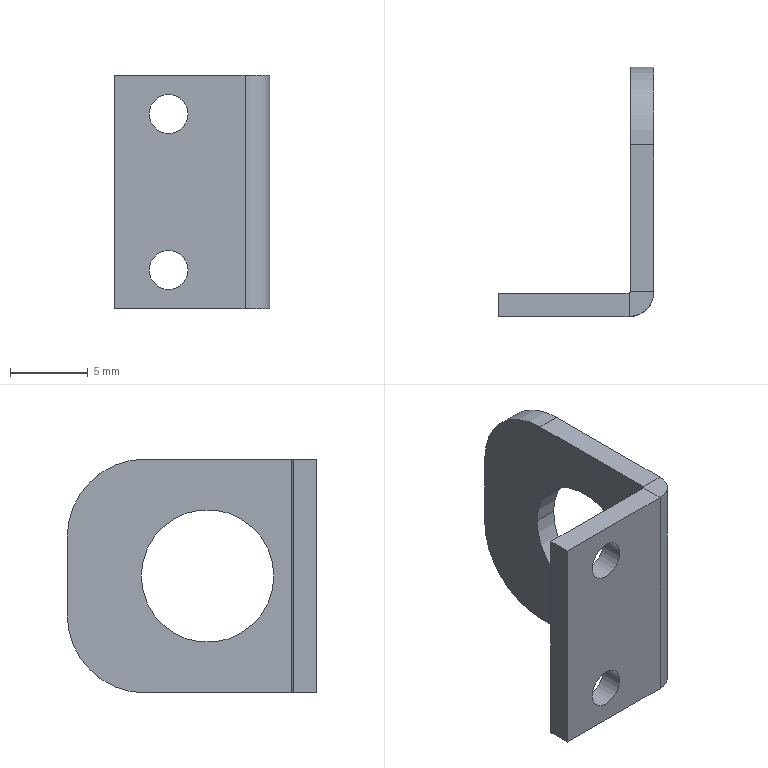Component | SolidWorks | FrontDoorAssembly-1_FrontDoorWelding-1_CustomLockBarGuidePlate-1 | 1 solid | 22 faces | box 10 x 16 x 15 mm | volume 427 mm3 | plane 12 | cylinder 10 | commonest cylinder face diameters 2.5 x4 8.5 x2 10 x2 3.2 x1 0.2 x1
STEP:
#1=CARTESIAN_POINT('',(-37.852,-11.035,14.951));
#2=VERTEX_POINT('',#1);
#3=CARTESIAN_POINT('',(-37.753,-11.035,14.951));
#4=VERTEX_POINT('',#3);
#5=CARTESIAN_POINT('',(-37.803,-11.035,14.951));
#6=DIRECTION('',(-0.,1.,-0.));
#7=DIRECTION('',(1.,0.,0.));
#8=AXIS2_PLACEMENT_3D('',#5,#6,#7);
#9=CIRCLE('',#8,0.04921);
#10=EDGE_CURVE('',#2,#4,#9,.T.);
#11=ORIENTED_EDGE('',*,*,#10,.F.);
#12=CARTESIAN_POINT('',(-37.852,-10.976,14.951));
#13=VERTEX_POINT('',#12);
#14=CARTESIAN_POINT('',(-37.852,-11.37,14.951));
#15=DIRECTION('',(-0.,1.,-0.));
#16=VECTOR('',#15,39.37);
#17=LINE('',#14,#16);
#18=EDGE_CURVE('',#2,#13,#17,.T.);
#19=ORIENTED_EDGE('',*,*,#18,.T.);
#20=CARTESIAN_POINT('',(-37.753,-10.976,14.951));
#21=VERTEX_POINT('',#20);
#22=CARTESIAN_POINT('',(-37.803,-10.976,14.951));
#23=DIRECTION('',(-0.,1.,-0.));
#24=DIRECTION('',(-1.,0.,0.));
#25=AXIS2_PLACEMENT_3D('',#22,#23,#24);
#26=CIRCLE('',#25,0.04921);
#27=EDGE_CURVE('',#13,#21,#26,.T.);
#28=ORIENTED_EDGE('',*,*,#27,.T.);
#29=CARTESIAN_POINT('',(-37.753,-11.37,14.951));
#30=DIRECTION('',(-0.,1.,-0.));
#31=VECTOR('',#30,39.37);
#32=LINE('',#29,#31);
#33=EDGE_CURVE('',#4,#21,#32,.T.);
#34=ORIENTED_EDGE('',*,*,#33,.F.);
#35=EDGE_LOOP('',(#11,#19,#28,#34));
#36=FACE_OUTER_BOUND('',#35,.T.);
#37=CARTESIAN_POINT('',(-37.803,-11.37,14.951));
#38=DIRECTION('',(-0.,1.,-0.));
#39=DIRECTION('',(1.,0.,0.));
#40=AXIS2_PLACEMENT_3D('',#37,#38,#39);
#41=CYLINDRICAL_SURFACE('',#40,0.04921);
#42=ADVANCED_FACE('',(#36),#41,.F.);
#43=CARTESIAN_POINT('',(-37.852,-11.035,14.557));
#44=VERTEX_POINT('',#43);
#45=CARTESIAN_POINT('',(-37.753,-11.035,14.557));
#46=VERTEX_POINT('',#45);
#47=CARTESIAN_POINT('',(-37.803,-11.035,14.557));
#48=DIRECTION('',(-0.,1.,-0.));
#49=DIRECTION('',(1.,0.,0.));
#50=AXIS2_PLACEMENT_3D('',#47,#48,#49);
#51=CIRCLE('',#50,0.04921);
#52=EDGE_CURVE('',#44,#46,#51,.T.);
#53=ORIENTED_EDGE('',*,*,#52,.F.);
#54=CARTESIAN_POINT('',(-37.852,-10.976,14.557));
#55=VERTEX_POINT('',#54);
#56=CARTESIAN_POINT('',(-37.852,-11.37,14.557));
#57=DIRECTION('',(-0.,1.,-0.));
#58=VECTOR('',#57,39.37);
#59=LINE('',#56,#58);
#60=EDGE_CURVE('',#44,#55,#59,.T.);
#61=ORIENTED_EDGE('',*,*,#60,.T.);
#62=CARTESIAN_POINT('',(-37.753,-10.976,14.557));
#63=VERTEX_POINT('',#62);
#64=CARTESIAN_POINT('',(-37.803,-10.976,14.557));
#65=DIRECTION('',(-0.,1.,-0.));
#66=DIRECTION('',(1.,0.,0.));
#67=AXIS2_PLACEMENT_3D('',#64,#65,#66);
#68=CIRCLE('',#67,0.04921);
#69=EDGE_CURVE('',#55,#63,#68,.T.);
#70=ORIENTED_EDGE('',*,*,#69,.T.);
#71=CARTESIAN_POINT('',(-37.753,-11.37,14.557));
#72=DIRECTION('',(-0.,1.,-0.));
#73=VECTOR('',#72,39.37);
#74=LINE('',#71,#73);
#75=EDGE_CURVE('',#46,#63,#74,.T.);
#76=ORIENTED_EDGE('',*,*,#75,.F.);
#77=EDGE_LOOP('',(#53,#61,#70,#76));
#78=FACE_OUTER_BOUND('',#77,.T.);
#79=CARTESIAN_POINT('',(-37.803,-11.37,14.557));
#80=DIRECTION('',(-0.,1.,-0.));
#81=DIRECTION('',(1.,0.,0.));
#82=AXIS2_PLACEMENT_3D('',#79,#80,#81);
#83=CYLINDRICAL_SURFACE('',#82,0.04921);
#84=ADVANCED_FACE('',(#78),#83,.F.);
#85=CARTESIAN_POINT('',(-37.547,-10.927,14.754));
#86=VERTEX_POINT('',#85);
#87=CARTESIAN_POINT('',(-37.547,-10.592,14.754));
#88=VERTEX_POINT('',#87);
#89=CARTESIAN_POINT('',(-37.547,-10.76,14.754));
#90=DIRECTION('',(-1.,0.,0.));
#91=DIRECTION('',(0.,1.,0.));
#92=AXIS2_PLACEMENT_3D('',#89,#90,#91);
#93=CIRCLE('',#92,0.1673);
#94=EDGE_CURVE('',#86,#88,#93,.T.);
#95=ORIENTED_EDGE('',*,*,#94,.F.);
#96=CARTESIAN_POINT('',(-37.606,-10.927,14.754));
#97=VERTEX_POINT('',#96);
#98=CARTESIAN_POINT('',(-37.212,-10.927,14.754));
#99=DIRECTION('',(-1.,0.,0.));
#100=VECTOR('',#99,39.37);
#101=LINE('',#98,#100);
#102=EDGE_CURVE('',#86,#97,#101,.T.);
#103=ORIENTED_EDGE('',*,*,#102,.T.);
#104=CARTESIAN_POINT('',(-37.606,-10.592,14.754));
#105=VERTEX_POINT('',#104);
#106=CARTESIAN_POINT('',(-37.606,-10.76,14.754));
#107=DIRECTION('',(-1.,0.,0.));
#108=DIRECTION('',(0.,1.,0.));
#109=AXIS2_PLACEMENT_3D('',#106,#107,#108);
#110=CIRCLE('',#109,0.1673);
#111=EDGE_CURVE('',#97,#105,#110,.T.);
#112=ORIENTED_EDGE('',*,*,#111,.T.);
#113=CARTESIAN_POINT('',(-37.212,-10.592,14.754));
#114=DIRECTION('',(-1.,0.,0.));
#115=VECTOR('',#114,39.37);
#116=LINE('',#113,#115);
#117=EDGE_CURVE('',#88,#105,#116,.T.);
#118=ORIENTED_EDGE('',*,*,#117,.F.);
#119=EDGE_LOOP('',(#95,#103,#112,#118));
#120=FACE_OUTER_BOUND('',#119,.T.);
#121=CARTESIAN_POINT('',(-37.212,-10.76,14.754));
#122=DIRECTION('',(-1.,0.,0.));
#123=DIRECTION('',(0.,1.,0.));
#124=AXIS2_PLACEMENT_3D('',#121,#122,#123);
#125=CYLINDRICAL_SURFACE('',#124,0.1673);
#126=ADVANCED_FACE('',(#120),#125,.F.);
#127=CARTESIAN_POINT('',(-37.547,-10.972,15.049));
#128=VERTEX_POINT('',#127);
#129=CARTESIAN_POINT('',(-37.547,-10.602,15.049));
#130=VERTEX_POINT('',#129);
#131=CARTESIAN_POINT('',(-37.547,-10.405,15.049));
#132=DIRECTION('',(0.,1.,-0.));
#133=VECTOR('',#132,39.37);
#134=LINE('',#131,#133);
#135=EDGE_CURVE('',#128,#130,#134,.T.);
#136=ORIENTED_EDGE('',*,*,#135,.T.);
#137=CARTESIAN_POINT('',(-37.606,-10.602,15.049));
#138=VERTEX_POINT('',#137);
#139=CARTESIAN_POINT('',(-37.547,-10.602,15.049));
#140=DIRECTION('',(-1.,0.,0.));
#141=VECTOR('',#140,39.37);
#142=LINE('',#139,#141);
#143=EDGE_CURVE('',#130,#138,#142,.T.);
#144=ORIENTED_EDGE('',*,*,#143,.T.);
#145=CARTESIAN_POINT('',(-37.606,-10.972,15.049));
#146=VERTEX_POINT('',#145);
#147=CARTESIAN_POINT('',(-37.606,-10.405,15.049));
#148=DIRECTION('',(0.,1.,-0.));
#149=VECTOR('',#148,39.37);
#150=LINE('',#147,#149);
#151=EDGE_CURVE('',#146,#138,#150,.T.);
#152=ORIENTED_EDGE('',*,*,#151,.F.);
#153=CARTESIAN_POINT('',(-37.606,-10.972,15.049));
#154=DIRECTION('',(1.,-0.,-0.));
#155=VECTOR('',#154,39.37);
#156=LINE('',#153,#155);
#157=EDGE_CURVE('',#146,#128,#156,.T.);
#158=ORIENTED_EDGE('',*,*,#157,.T.);
#159=EDGE_LOOP('',(#136,#144,#152,#158));
#160=FACE_OUTER_BOUND('',#159,.T.);
#161=CARTESIAN_POINT('',(-37.547,-10.405,15.049));
#162=DIRECTION('',(0.,0.,1.));
#163=DIRECTION('',(0.,1.,-0.));
#164=AXIS2_PLACEMENT_3D('',#161,#162,#163);
#165=PLANE('',#164);
#166=ADVANCED_FACE('',(#160),#165,.T.);
#167=CARTESIAN_POINT('',(-37.547,-10.76,14.754));
#168=DIRECTION('',(-1.,0.,0.));
#169=DIRECTION('',(0.,1.,0.));
#170=AXIS2_PLACEMENT_3D('',#167,#168,#169);
#171=CIRCLE('',#170,0.1673);
#172=EDGE_CURVE('',#88,#86,#171,.T.);
#173=ORIENTED_EDGE('',*,*,#172,.T.);
#174=ORIENTED_EDGE('',*,*,#94,.T.);
#175=EDGE_LOOP('',(#173,#174));
#176=FACE_BOUND('',#175,.T.);
#177=CARTESIAN_POINT('',(-37.547,-10.405,14.853));
#178=VERTEX_POINT('',#177);
#179=CARTESIAN_POINT('',(-37.547,-10.405,14.656));
#180=VERTEX_POINT('',#179);
#181=CARTESIAN_POINT('',(-37.547,-10.405,15.049));
#182=DIRECTION('',(-0.,-0.,-1.));
#183=VECTOR('',#182,39.37);
#184=LINE('',#181,#183);
#185=EDGE_CURVE('',#178,#180,#184,.T.);
#186=ORIENTED_EDGE('',*,*,#185,.F.);
#187=CARTESIAN_POINT('',(-37.547,-10.602,14.853));
#188=DIRECTION('',(1.,-0.,-0.));
#189=DIRECTION('',(0.,1.,0.));
#190=AXIS2_PLACEMENT_3D('',#187,#188,#189);
#191=CIRCLE('',#190,0.1969);
#192=EDGE_CURVE('',#178,#130,#191,.T.);
#193=ORIENTED_EDGE('',*,*,#192,.T.);
#194=ORIENTED_EDGE('',*,*,#135,.F.);
#195=CARTESIAN_POINT('',(-37.547,-10.972,14.459));
#196=VERTEX_POINT('',#195);
#197=CARTESIAN_POINT('',(-37.547,-10.972,15.049));
#198=DIRECTION('',(-0.,-0.,-1.));
#199=VECTOR('',#198,39.37);
#200=LINE('',#197,#199);
#201=EDGE_CURVE('',#128,#196,#200,.T.);
#202=ORIENTED_EDGE('',*,*,#201,.T.);
#203=CARTESIAN_POINT('',(-37.547,-10.602,14.459));
#204=VERTEX_POINT('',#203);
#205=CARTESIAN_POINT('',(-37.547,-10.405,14.459));
#206=DIRECTION('',(-0.,-1.,0.));
#207=VECTOR('',#206,39.37);
#208=LINE('',#205,#207);
#209=EDGE_CURVE('',#204,#196,#208,.T.);
#210=ORIENTED_EDGE('',*,*,#209,.F.);
#211=CARTESIAN_POINT('',(-37.547,-10.602,14.656));
#212=DIRECTION('',(1.,-0.,-0.));
#213=DIRECTION('',(0.,1.,0.));
#214=AXIS2_PLACEMENT_3D('',#211,#212,#213);
#215=CIRCLE('',#214,0.1969);
#216=EDGE_CURVE('',#204,#180,#215,.T.);
#217=ORIENTED_EDGE('',*,*,#216,.T.);
#218=EDGE_LOOP('',(#186,#193,#194,#202,#210,#217));
#219=FACE_OUTER_BOUND('',#218,.T.);
#220=CARTESIAN_POINT('',(-37.547,-10.72,14.754));
#221=DIRECTION('',(-1.,0.,0.));
#222=DIRECTION('',(0.,1.,-0.));
#223=AXIS2_PLACEMENT_3D('',#220,#221,#222);
#224=PLANE('',#223);
#225=ADVANCED_FACE('',(#176,#219),#224,.F.);
#226=CARTESIAN_POINT('',(-37.606,-10.76,14.754));
#227=DIRECTION('',(-1.,0.,0.));
#228=DIRECTION('',(0.,1.,0.));
#229=AXIS2_PLACEMENT_3D('',#226,#227,#228);
#230=CIRCLE('',#229,0.1673);
#231=EDGE_CURVE('',#105,#97,#230,.T.);
#232=ORIENTED_EDGE('',*,*,#231,.F.);
#233=ORIENTED_EDGE('',*,*,#111,.F.);
#234=EDGE_LOOP('',(#232,#233));
#235=FACE_BOUND('',#234,.T.);
#236=ORIENTED_EDGE('',*,*,#151,.T.);
#237=CARTESIAN_POINT('',(-37.606,-10.405,14.853));
#238=VERTEX_POINT('',#237);
#239=CARTESIAN_POINT('',(-37.606,-10.602,14.853));
#240=DIRECTION('',(-1.,0.,0.));
#241=DIRECTION('',(0.,1.,0.));
#242=AXIS2_PLACEMENT_3D('',#239,#240,#241);
#243=CIRCLE('',#242,0.1969);
#244=EDGE_CURVE('',#138,#238,#243,.T.);
#245=ORIENTED_EDGE('',*,*,#244,.T.);
#246=CARTESIAN_POINT('',(-37.606,-10.405,14.656));
#247=VERTEX_POINT('',#246);
#248=CARTESIAN_POINT('',(-37.606,-10.405,15.049));
#249=DIRECTION('',(-0.,-0.,-1.));
#250=VECTOR('',#249,39.37);
#251=LINE('',#248,#250);
#252=EDGE_CURVE('',#238,#247,#251,.T.);
#253=ORIENTED_EDGE('',*,*,#252,.T.);
#254=CARTESIAN_POINT('',(-37.606,-10.602,14.459));
#255=VERTEX_POINT('',#254);
#256=CARTESIAN_POINT('',(-37.606,-10.602,14.656));
#257=DIRECTION('',(-1.,0.,0.));
#258=DIRECTION('',(0.,1.,0.));
#259=AXIS2_PLACEMENT_3D('',#256,#257,#258);
#260=CIRCLE('',#259,0.1969);
#261=EDGE_CURVE('',#247,#255,#260,.T.);
#262=ORIENTED_EDGE('',*,*,#261,.T.);
#263=CARTESIAN_POINT('',(-37.606,-10.972,14.459));
#264=VERTEX_POINT('',#263);
#265=CARTESIAN_POINT('',(-37.606,-10.405,14.459));
#266=DIRECTION('',(-0.,-1.,0.));
#267=VECTOR('',#266,39.37);
#268=LINE('',#265,#267);
#269=EDGE_CURVE('',#255,#264,#268,.T.);
#270=ORIENTED_EDGE('',*,*,#269,.T.);
#271=CARTESIAN_POINT('',(-37.606,-10.972,15.049));
#272=DIRECTION('',(-0.,-0.,-1.));
#273=VECTOR('',#272,39.37);
#274=LINE('',#271,#273);
#275=EDGE_CURVE('',#146,#264,#274,.T.);
#276=ORIENTED_EDGE('',*,*,#275,.F.);
#277=EDGE_LOOP('',(#236,#245,#253,#262,#270,#276));
#278=FACE_OUTER_BOUND('',#277,.T.);
#279=CARTESIAN_POINT('',(-37.606,-10.72,14.754));
#280=DIRECTION('',(-1.,0.,0.));
#281=DIRECTION('',(0.,1.,-0.));
#282=AXIS2_PLACEMENT_3D('',#279,#280,#281);
#283=PLANE('',#282);
#284=ADVANCED_FACE('',(#235,#278),#283,.T.);
#285=ORIENTED_EDGE('',*,*,#269,.F.);
#286=CARTESIAN_POINT('',(-37.547,-10.602,14.459));
#287=DIRECTION('',(1.,-0.,-0.));
#288=VECTOR('',#287,39.37);
#289=LINE('',#286,#288);
#290=EDGE_CURVE('',#255,#204,#289,.T.);
#291=ORIENTED_EDGE('',*,*,#290,.T.);
#292=ORIENTED_EDGE('',*,*,#209,.T.);
#293=CARTESIAN_POINT('',(-37.606,-10.972,14.459));
#294=DIRECTION('',(1.,-0.,-0.));
#295=VECTOR('',#294,39.37);
#296=LINE('',#293,#295);
#297=EDGE_CURVE('',#264,#196,#296,.T.);
#298=ORIENTED_EDGE('',*,*,#297,.F.);
#299=EDGE_LOOP('',(#285,#291,#292,#298));
#300=FACE_OUTER_BOUND('',#299,.T.);
#301=CARTESIAN_POINT('',(-37.547,-10.405,14.459));
#302=DIRECTION('',(-0.,-0.,-1.));
#303=DIRECTION('',(-0.,-1.,0.));
#304=AXIS2_PLACEMENT_3D('',#301,#302,#303);
#305=PLANE('',#304);
#306=ADVANCED_FACE('',(#300),#305,.T.);
#307=ORIENTED_EDGE('',*,*,#252,.F.);
#308=CARTESIAN_POINT('',(-37.547,-10.405,14.853));
#309=DIRECTION('',(1.,-0.,-0.));
#310=VECTOR('',#309,39.37);
#311=LINE('',#308,#310);
#312=EDGE_CURVE('',#238,#178,#311,.T.);
#313=ORIENTED_EDGE('',*,*,#312,.T.);
#314=ORIENTED_EDGE('',*,*,#185,.T.);
#315=CARTESIAN_POINT('',(-37.547,-10.405,14.656));
#316=DIRECTION('',(-1.,0.,0.));
#317=VECTOR('',#316,39.37);
#318=LINE('',#315,#317);
#319=EDGE_CURVE('',#180,#247,#318,.T.);
#320=ORIENTED_EDGE('',*,*,#319,.T.);
#321=EDGE_LOOP('',(#307,#313,#314,#320));
#322=FACE_OUTER_BOUND('',#321,.T.);
#323=CARTESIAN_POINT('',(-37.547,-10.405,15.049));
#324=DIRECTION('',(0.,1.,-0.));
#325=DIRECTION('',(1.,-0.,-0.));
#326=AXIS2_PLACEMENT_3D('',#323,#324,#325);
#327=PLANE('',#326);
#328=ADVANCED_FACE('',(#322),#327,.T.);
#329=CARTESIAN_POINT('',(-37.61,-10.976,14.459));
#330=VERTEX_POINT('',#329);
#331=CARTESIAN_POINT('',(-37.61,-11.035,14.459));
#332=VERTEX_POINT('',#331);
#333=CARTESIAN_POINT('',(-37.61,-11.035,14.459));
#334=DIRECTION('',(0.,-1.,0.));
#335=VECTOR('',#334,39.37);
#336=LINE('',#333,#335);
#337=EDGE_CURVE('',#330,#332,#336,.T.);
#338=ORIENTED_EDGE('',*,*,#337,.F.);
#339=CARTESIAN_POINT('',(-37.61,-10.972,14.459));
#340=DIRECTION('',(-0.,-0.,-1.));
#341=DIRECTION('',(1.,0.,0.));
#342=AXIS2_PLACEMENT_3D('',#339,#340,#341);
#343=CIRCLE('',#342,0.003937);
#344=EDGE_CURVE('',#264,#330,#343,.T.);
#345=ORIENTED_EDGE('',*,*,#344,.F.);
#346=ORIENTED_EDGE('',*,*,#297,.T.);
#347=CARTESIAN_POINT('',(-37.61,-10.972,14.459));
#348=DIRECTION('',(-0.,-0.,-1.));
#349=DIRECTION('',(1.,0.,0.));
#350=AXIS2_PLACEMENT_3D('',#347,#348,#349);
#351=CIRCLE('',#350,0.06299);
#352=EDGE_CURVE('',#196,#332,#351,.T.);
#353=ORIENTED_EDGE('',*,*,#352,.T.);
#354=EDGE_LOOP('',(#338,#345,#346,#353));
#355=FACE_OUTER_BOUND('',#354,.T.);
#356=CARTESIAN_POINT('',(-37.61,-10.972,14.459));
#357=DIRECTION('',(-0.,0.,-1.));
#358=DIRECTION('',(-1.,0.,0.));
#359=AXIS2_PLACEMENT_3D('',#356,#357,#358);
#360=PLANE('',#359);
#361=ADVANCED_FACE('',(#355),#360,.T.);
#362=CARTESIAN_POINT('',(-37.61,-10.976,15.049));
#363=VERTEX_POINT('',#362);
#364=CARTESIAN_POINT('',(-37.61,-10.972,15.049));
#365=DIRECTION('',(0.,0.,1.));
#366=DIRECTION('',(1.,0.,0.));
#367=AXIS2_PLACEMENT_3D('',#364,#365,#366);
#368=CIRCLE('',#367,0.003937);
#369=EDGE_CURVE('',#363,#146,#368,.T.);
#370=ORIENTED_EDGE('',*,*,#369,.F.);
#371=CARTESIAN_POINT('',(-37.61,-11.035,15.049));
#372=VERTEX_POINT('',#371);
#373=CARTESIAN_POINT('',(-37.61,-10.976,15.049));
#374=DIRECTION('',(0.,-1.,0.));
#375=VECTOR('',#374,39.37);
#376=LINE('',#373,#375);
#377=EDGE_CURVE('',#363,#372,#376,.T.);
#378=ORIENTED_EDGE('',*,*,#377,.T.);
#379=CARTESIAN_POINT('',(-37.61,-10.972,15.049));
#380=DIRECTION('',(0.,0.,1.));
#381=DIRECTION('',(1.,0.,0.));
#382=AXIS2_PLACEMENT_3D('',#379,#380,#381);
#383=CIRCLE('',#382,0.06299);
#384=EDGE_CURVE('',#372,#128,#383,.T.);
#385=ORIENTED_EDGE('',*,*,#384,.T.);
#386=ORIENTED_EDGE('',*,*,#157,.F.);
#387=EDGE_LOOP('',(#370,#378,#385,#386));
#388=FACE_OUTER_BOUND('',#387,.T.);
#389=CARTESIAN_POINT('',(-37.61,-10.972,15.049));
#390=DIRECTION('',(-0.,0.,-1.));
#391=DIRECTION('',(-1.,0.,0.));
#392=AXIS2_PLACEMENT_3D('',#389,#390,#391);
#393=PLANE('',#392);
#394=ADVANCED_FACE('',(#388),#393,.F.);
#395=ORIENTED_EDGE('',*,*,#201,.F.);
#396=ORIENTED_EDGE('',*,*,#384,.F.);
#397=CARTESIAN_POINT('',(-37.61,-11.035,14.459));
#398=DIRECTION('',(-0.,-0.,-1.));
#399=VECTOR('',#398,39.37);
#400=LINE('',#397,#399);
#401=EDGE_CURVE('',#372,#332,#400,.T.);
#402=ORIENTED_EDGE('',*,*,#401,.T.);
#403=ORIENTED_EDGE('',*,*,#352,.F.);
#404=EDGE_LOOP('',(#395,#396,#402,#403));
#405=FACE_OUTER_BOUND('',#404,.T.);
#406=CARTESIAN_POINT('',(-37.61,-10.972,15.049));
#407=DIRECTION('',(0.,0.,1.));
#408=DIRECTION('',(0.,-1.,0.));
#409=AXIS2_PLACEMENT_3D('',#406,#407,#408);
#410=CYLINDRICAL_SURFACE('',#409,0.06299);
#411=ADVANCED_FACE('',(#405),#410,.T.);
#412=ORIENTED_EDGE('',*,*,#275,.T.);
#413=ORIENTED_EDGE('',*,*,#344,.T.);
#414=CARTESIAN_POINT('',(-37.61,-10.976,14.459));
#415=DIRECTION('',(0.,0.,1.));
#416=VECTOR('',#415,39.37);
#417=LINE('',#414,#416);
#418=EDGE_CURVE('',#330,#363,#417,.T.);
#419=ORIENTED_EDGE('',*,*,#418,.T.);
#420=ORIENTED_EDGE('',*,*,#369,.T.);
#421=EDGE_LOOP('',(#412,#413,#419,#420));
#422=FACE_OUTER_BOUND('',#421,.T.);
#423=CARTESIAN_POINT('',(-37.61,-10.972,15.049));
#424=DIRECTION('',(0.,0.,1.));
#425=DIRECTION('',(0.,-1.,0.));
#426=AXIS2_PLACEMENT_3D('',#423,#424,#425);
#427=CYLINDRICAL_SURFACE('',#426,0.003937);
#428=ADVANCED_FACE('',(#422),#427,.F.);
#429=ORIENTED_EDGE('',*,*,#337,.T.);
#430=CARTESIAN_POINT('',(-37.94,-11.035,14.459));
#431=VERTEX_POINT('',#430);
#432=CARTESIAN_POINT('',(-37.606,-11.035,14.459));
#433=DIRECTION('',(1.,0.,-0.));
#434=VECTOR('',#433,39.37);
#435=LINE('',#432,#434);
#436=EDGE_CURVE('',#431,#332,#435,.T.);
#437=ORIENTED_EDGE('',*,*,#436,.F.);
#438=CARTESIAN_POINT('',(-37.94,-10.976,14.459));
#439=VERTEX_POINT('',#438);
#440=CARTESIAN_POINT('',(-37.94,-11.035,14.459));
#441=DIRECTION('',(-0.,1.,-0.));
#442=VECTOR('',#441,39.37);
#443=LINE('',#440,#442);
#444=EDGE_CURVE('',#431,#439,#443,.T.);
#445=ORIENTED_EDGE('',*,*,#444,.T.);
#446=CARTESIAN_POINT('',(-37.606,-10.976,14.459));
#447=DIRECTION('',(1.,0.,-0.));
#448=VECTOR('',#447,39.37);
#449=LINE('',#446,#448);
#450=EDGE_CURVE('',#439,#330,#449,.T.);
#451=ORIENTED_EDGE('',*,*,#450,.T.);
#452=EDGE_LOOP('',(#429,#437,#445,#451));
#453=FACE_OUTER_BOUND('',#452,.T.);
#454=CARTESIAN_POINT('',(-37.606,-11.035,14.459));
#455=DIRECTION('',(0.,-0.,1.));
#456=DIRECTION('',(1.,-0.,-0.));
#457=AXIS2_PLACEMENT_3D('',#454,#455,#456);
#458=PLANE('',#457);
#459=ADVANCED_FACE('',(#453),#458,.F.);
#460=ORIENTED_EDGE('',*,*,#377,.F.);
#461=CARTESIAN_POINT('',(-37.94,-10.976,15.049));
#462=VERTEX_POINT('',#461);
#463=CARTESIAN_POINT('',(-37.94,-10.976,15.049));
#464=DIRECTION('',(-1.,-0.,0.));
#465=VECTOR('',#464,39.37);
#466=LINE('',#463,#465);
#467=EDGE_CURVE('',#363,#462,#466,.T.);
#468=ORIENTED_EDGE('',*,*,#467,.T.);
#469=CARTESIAN_POINT('',(-37.94,-11.035,15.049));
#470=VERTEX_POINT('',#469);
#471=CARTESIAN_POINT('',(-37.94,-11.035,15.049));
#472=DIRECTION('',(-0.,1.,-0.));
#473=VECTOR('',#472,39.37);
#474=LINE('',#471,#473);
#475=EDGE_CURVE('',#470,#462,#474,.T.);
#476=ORIENTED_EDGE('',*,*,#475,.F.);
#477=CARTESIAN_POINT('',(-37.606,-11.035,15.049));
#478=DIRECTION('',(-1.,-0.,0.));
#479=VECTOR('',#478,39.37);
#480=LINE('',#477,#479);
#481=EDGE_CURVE('',#372,#470,#480,.T.);
#482=ORIENTED_EDGE('',*,*,#481,.F.);
#483=EDGE_LOOP('',(#460,#468,#476,#482));
#484=FACE_OUTER_BOUND('',#483,.T.);
#485=CARTESIAN_POINT('',(-37.94,-11.035,15.049));
#486=DIRECTION('',(-0.,0.,-1.));
#487=DIRECTION('',(-1.,0.,0.));
#488=AXIS2_PLACEMENT_3D('',#485,#486,#487);
#489=PLANE('',#488);
#490=ADVANCED_FACE('',(#484),#489,.F.);
#491=CARTESIAN_POINT('',(-37.803,-11.035,14.951));
#492=DIRECTION('',(-0.,1.,-0.));
#493=DIRECTION('',(1.,0.,0.));
#494=AXIS2_PLACEMENT_3D('',#491,#492,#493);
#495=CIRCLE('',#494,0.04921);
#496=EDGE_CURVE('',#4,#2,#495,.T.);
#497=ORIENTED_EDGE('',*,*,#496,.T.);
#498=ORIENTED_EDGE('',*,*,#10,.T.);
#499=EDGE_LOOP('',(#497,#498));
#500=FACE_BOUND('',#499,.T.);
#501=CARTESIAN_POINT('',(-37.803,-11.035,14.557));
#502=DIRECTION('',(-0.,1.,-0.));
#503=DIRECTION('',(1.,0.,0.));
#504=AXIS2_PLACEMENT_3D('',#501,#502,#503);
#505=CIRCLE('',#504,0.04921);
#506=EDGE_CURVE('',#46,#44,#505,.T.);
#507=ORIENTED_EDGE('',*,*,#506,.T.);
#508=ORIENTED_EDGE('',*,*,#52,.T.);
#509=EDGE_LOOP('',(#507,#508));
#510=FACE_BOUND('',#509,.T.);
#511=ORIENTED_EDGE('',*,*,#401,.F.);
#512=ORIENTED_EDGE('',*,*,#481,.T.);
#513=CARTESIAN_POINT('',(-37.94,-11.035,14.754));
#514=DIRECTION('',(-0.,-0.,-1.));
#515=VECTOR('',#514,39.37);
#516=LINE('',#513,#515);
#517=EDGE_CURVE('',#470,#431,#516,.T.);
#518=ORIENTED_EDGE('',*,*,#517,.T.);
#519=ORIENTED_EDGE('',*,*,#436,.T.);
#520=EDGE_LOOP('',(#511,#512,#518,#519));
#521=FACE_OUTER_BOUND('',#520,.T.);
#522=CARTESIAN_POINT('',(-37.606,-11.035,14.754));
#523=DIRECTION('',(-0.,1.,-0.));
#524=DIRECTION('',(1.,0.,-0.));
#525=AXIS2_PLACEMENT_3D('',#522,#523,#524);
#526=PLANE('',#525);
#527=ADVANCED_FACE('',(#500,#510,#521),#526,.F.);
#528=CARTESIAN_POINT('',(-37.803,-10.976,14.951));
#529=DIRECTION('',(-0.,1.,-0.));
#530=DIRECTION('',(-1.,0.,0.));
#531=AXIS2_PLACEMENT_3D('',#528,#529,#530);
#532=CIRCLE('',#531,0.04921);
#533=EDGE_CURVE('',#21,#13,#532,.T.);
#534=ORIENTED_EDGE('',*,*,#533,.F.);
#535=ORIENTED_EDGE('',*,*,#27,.F.);
#536=EDGE_LOOP('',(#534,#535));
#537=FACE_BOUND('',#536,.T.);
#538=CARTESIAN_POINT('',(-37.803,-10.976,14.557));
#539=DIRECTION('',(-0.,1.,-0.));
#540=DIRECTION('',(1.,0.,0.));
#541=AXIS2_PLACEMENT_3D('',#538,#539,#540);
#542=CIRCLE('',#541,0.04921);
#543=EDGE_CURVE('',#63,#55,#542,.T.);
#544=ORIENTED_EDGE('',*,*,#543,.F.);
#545=ORIENTED_EDGE('',*,*,#69,.F.);
#546=EDGE_LOOP('',(#544,#545));
#547=FACE_BOUND('',#546,.T.);
#548=ORIENTED_EDGE('',*,*,#467,.F.);
#549=ORIENTED_EDGE('',*,*,#418,.F.);
#550=ORIENTED_EDGE('',*,*,#450,.F.);
#551=CARTESIAN_POINT('',(-37.94,-10.976,14.459));
#552=DIRECTION('',(-0.,-0.,-1.));
#553=VECTOR('',#552,39.37);
#554=LINE('',#551,#553);
#555=EDGE_CURVE('',#462,#439,#554,.T.);
#556=ORIENTED_EDGE('',*,*,#555,.F.);
#557=EDGE_LOOP('',(#548,#549,#550,#556));
#558=FACE_OUTER_BOUND('',#557,.T.);
#559=CARTESIAN_POINT('',(-37.606,-10.976,14.754));
#560=DIRECTION('',(-0.,1.,-0.));
#561=DIRECTION('',(1.,0.,-0.));
#562=AXIS2_PLACEMENT_3D('',#559,#560,#561);
#563=PLANE('',#562);
#564=ADVANCED_FACE('',(#537,#547,#558),#563,.T.);
#565=ORIENTED_EDGE('',*,*,#555,.T.);
#566=ORIENTED_EDGE('',*,*,#444,.F.);
#567=ORIENTED_EDGE('',*,*,#517,.F.);
#568=ORIENTED_EDGE('',*,*,#475,.T.);
#569=EDGE_LOOP('',(#565,#566,#567,#568));
#570=FACE_OUTER_BOUND('',#569,.T.);
#571=CARTESIAN_POINT('',(-37.94,-11.035,14.459));
#572=DIRECTION('',(1.,0.,-0.));
#573=DIRECTION('',(0.,-1.,0.));
#574=AXIS2_PLACEMENT_3D('',#571,#572,#573);
#575=PLANE('',#574);
#576=ADVANCED_FACE('',(#570),#575,.F.);
#577=ORIENTED_EDGE('',*,*,#102,.F.);
#578=ORIENTED_EDGE('',*,*,#172,.F.);
#579=ORIENTED_EDGE('',*,*,#117,.T.);
#580=ORIENTED_EDGE('',*,*,#231,.T.);
#581=EDGE_LOOP('',(#577,#578,#579,#580));
#582=FACE_OUTER_BOUND('',#581,.T.);
#583=CARTESIAN_POINT('',(-37.212,-10.76,14.754));
#584=DIRECTION('',(-1.,0.,0.));
#585=DIRECTION('',(0.,1.,0.));
#586=AXIS2_PLACEMENT_3D('',#583,#584,#585);
#587=CYLINDRICAL_SURFACE('',#586,0.1673);
#588=ADVANCED_FACE('',(#582),#587,.F.);
#589=ORIENTED_EDGE('',*,*,#192,.F.);
#590=ORIENTED_EDGE('',*,*,#312,.F.);
#591=ORIENTED_EDGE('',*,*,#244,.F.);
#592=ORIENTED_EDGE('',*,*,#143,.F.);
#593=EDGE_LOOP('',(#589,#590,#591,#592));
#594=FACE_OUTER_BOUND('',#593,.T.);
#595=CARTESIAN_POINT('',(-37.547,-10.602,14.853));
#596=DIRECTION('',(-1.,0.,0.));
#597=DIRECTION('',(0.,1.,0.));
#598=AXIS2_PLACEMENT_3D('',#595,#596,#597);
#599=CYLINDRICAL_SURFACE('',#598,0.1969);
#600=ADVANCED_FACE('',(#594),#599,.T.);
#601=ORIENTED_EDGE('',*,*,#216,.F.);
#602=ORIENTED_EDGE('',*,*,#290,.F.);
#603=ORIENTED_EDGE('',*,*,#261,.F.);
#604=ORIENTED_EDGE('',*,*,#319,.F.);
#605=EDGE_LOOP('',(#601,#602,#603,#604));
#606=FACE_OUTER_BOUND('',#605,.T.);
#607=CARTESIAN_POINT('',(-37.547,-10.602,14.656));
#608=DIRECTION('',(-1.,0.,0.));
#609=DIRECTION('',(0.,1.,0.));
#610=AXIS2_PLACEMENT_3D('',#607,#608,#609);
#611=CYLINDRICAL_SURFACE('',#610,0.1969);
#612=ADVANCED_FACE('',(#606),#611,.T.);
#613=ORIENTED_EDGE('',*,*,#60,.F.);
#614=ORIENTED_EDGE('',*,*,#506,.F.);
#615=ORIENTED_EDGE('',*,*,#75,.T.);
#616=ORIENTED_EDGE('',*,*,#543,.T.);
#617=EDGE_LOOP('',(#613,#614,#615,#616));
#618=FACE_OUTER_BOUND('',#617,.T.);
#619=CARTESIAN_POINT('',(-37.803,-11.37,14.557));
#620=DIRECTION('',(-0.,1.,-0.));
#621=DIRECTION('',(1.,0.,0.));
#622=AXIS2_PLACEMENT_3D('',#619,#620,#621);
#623=CYLINDRICAL_SURFACE('',#622,0.04921);
#624=ADVANCED_FACE('',(#618),#623,.F.);
#625=ORIENTED_EDGE('',*,*,#18,.F.);
#626=ORIENTED_EDGE('',*,*,#496,.F.);
#627=ORIENTED_EDGE('',*,*,#33,.T.);
#628=ORIENTED_EDGE('',*,*,#533,.T.);
#629=EDGE_LOOP('',(#625,#626,#627,#628));
#630=FACE_OUTER_BOUND('',#629,.T.);
#631=CARTESIAN_POINT('',(-37.803,-11.37,14.951));
#632=DIRECTION('',(-0.,1.,-0.));
#633=DIRECTION('',(1.,0.,0.));
#634=AXIS2_PLACEMENT_3D('',#631,#632,#633);
#635=CYLINDRICAL_SURFACE('',#634,0.04921);
#636=ADVANCED_FACE('',(#630),#635,.F.);
#637=CLOSED_SHELL('',(#42,#84,#126,#166,#225,#284,#306,#328,#361,#394,#411,#428,#459,#490,#527,#564,#576,#588,#600,#612,#624,#636));
#638=MANIFOLD_SOLID_BREP('',#637);
#639=CARTESIAN_POINT('',(0.,0.,0.));
#640=DIRECTION('',(0.,0.,1.));
#641=DIRECTION('',(1.,0.,0.));
#642=AXIS2_PLACEMENT_3D('',#639,#640,#641);
#643=(LENGTH_UNIT()NAMED_UNIT(*)SI_UNIT($,.METRE.));
#644=LENGTH_MEASURE_WITH_UNIT(LENGTH_MEASURE(0.0254),#643);
#645=DIMENSIONAL_EXPONENTS(1.,0.,0.,0.,0.,0.,0.);
#646=(CONVERSION_BASED_UNIT('',#644)LENGTH_UNIT()NAMED_UNIT(#645));
#647=UNCERTAINTY_MEASURE_WITH_UNIT(LENGTH_MEASURE(0.00001),#646,'','');
#648=(NAMED_UNIT(*)PLANE_ANGLE_UNIT()SI_UNIT($,.RADIAN.));
#649=(NAMED_UNIT(*)SI_UNIT($,.STERADIAN.)SOLID_ANGLE_UNIT());
#650=(GEOMETRIC_REPRESENTATION_CONTEXT(3)GLOBAL_UNCERTAINTY_ASSIGNED_CONTEXT((#647))GLOBAL_UNIT_ASSIGNED_CONTEXT((#646,#648,#649))REPRESENTATION_CONTEXT('',''));
#651=ADVANCED_BREP_SHAPE_REPRESENTATION('',(#638,#642),#650);
#652=COLOUR_RGB('',0.7922,0.8196,0.9333);
#653=FILL_AREA_STYLE_COLOUR('',#652);
#654=FILL_AREA_STYLE('',(#653));
#655=SURFACE_STYLE_FILL_AREA(#654);
#656=SURFACE_SIDE_STYLE('',(#655));
#657=SURFACE_STYLE_USAGE(.BOTH.,#656);
#658=PRESENTATION_STYLE_ASSIGNMENT((#657));
#659=STYLED_ITEM('',(#658),#638);
#660=(LENGTH_UNIT()NAMED_UNIT(*)SI_UNIT($,.METRE.));
#661=LENGTH_MEASURE_WITH_UNIT(LENGTH_MEASURE(0.0254),#660);
#662=DIMENSIONAL_EXPONENTS(1.,0.,0.,0.,0.,0.,0.);
#663=(CONVERSION_BASED_UNIT('',#661)LENGTH_UNIT()NAMED_UNIT(#662));
#664=UNCERTAINTY_MEASURE_WITH_UNIT(LENGTH_MEASURE(0.00001),#663,'','');
#665=(NAMED_UNIT(*)PLANE_ANGLE_UNIT()SI_UNIT($,.RADIAN.));
#666=(NAMED_UNIT(*)SI_UNIT($,.STERADIAN.)SOLID_ANGLE_UNIT());
#667=(GEOMETRIC_REPRESENTATION_CONTEXT(3)GLOBAL_UNCERTAINTY_ASSIGNED_CONTEXT((#664))GLOBAL_UNIT_ASSIGNED_CONTEXT((#663,#665,#666))REPRESENTATION_CONTEXT('',''));
#668=MECHANICAL_DESIGN_GEOMETRIC_PRESENTATION_REPRESENTATION('',(#659),#667);
#669=PRESENTATION_LAYER_ASSIGNMENT('','',(#659));